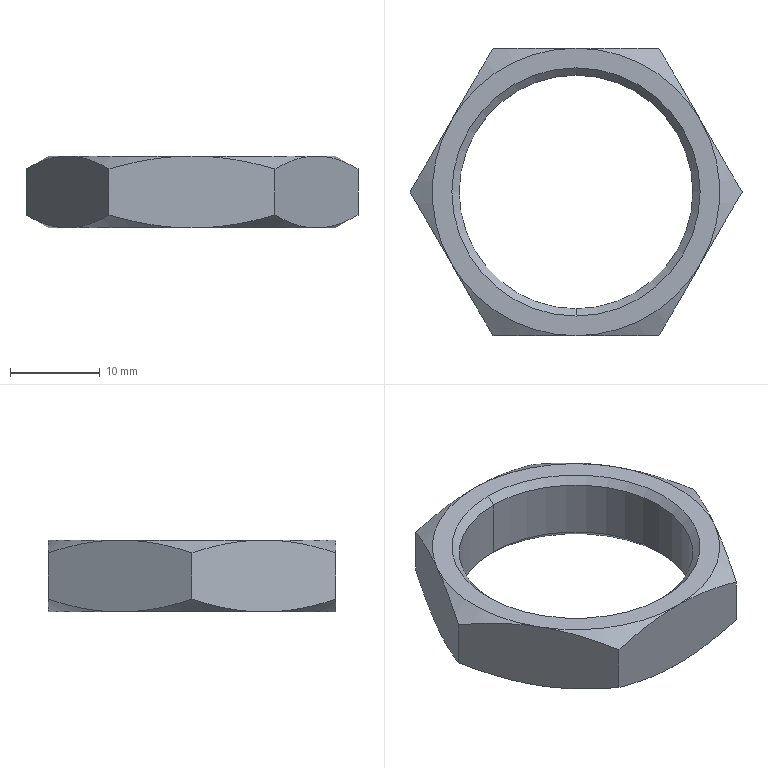Component | SolidWorks | MF_25x50_S_U_M_2_0-1_MF25_M26x1_5_Nut-1 | 1 solid | 26 faces | box 36.95 x 32 x 8 mm | volume 2721 mm3 | cone 16 | plane 8 | cylinder 2 | commonest cylinder face diameters 26 x2
build123d program:
from build123d import *

# Parameters (mm, degrees)
SKETCH2_W      = 64
SKETCH2_H      = 64
EXTRUDE1_DEPTH = 8


with BuildPart() as part:
    # Sketch1 → Revolve1 (revolve)
    with BuildSketch(Plane.XY, mode=Mode.PRIVATE) as revolve1_sk:
        Polygon((0, 0), (0, 16), (1.848, 19.2), (6.152, 19.2), (8, 16), (8, 0), align=None)
    revolve(revolve1_sk.sketch.rotate(Axis((8, 0, 0), (-1, 0, 0)), 270), axis=Axis((8, 0, 0), (-1, 0, 0)))

    # Sketch2 → Extrude1 (cut)
    with BuildSketch(Plane(origin=(0, 0, 0), x_dir=(0, 0, -1), z_dir=(1, 0, 0))):
        Rectangle(SKETCH2_W, SKETCH2_H)
        Polygon((-16, 9.238), (-16, -9.238), (0, -18.475), (16, -9.238), (16, 9.238), (0, 18.475), align=None, mode=Mode.SUBTRACT)
    extrude(amount=EXTRUDE1_DEPTH, mode=Mode.SUBTRACT)

    # Sketch3 → Cut-Revolve1 (revolve, cut)
    with BuildSketch(Plane.XY, mode=Mode.PRIVATE) as cut_revolve1_sk:
        Polygon((0, 0), (0, 13), (0.812, 12.188), (7.188, 12.188), (8, 13), (8, 0), align=None)
    revolve(cut_revolve1_sk.sketch.rotate(Axis((8, 0, 0), (-1, 0, 0)), 270), axis=Axis((8, 0, 0), (-1, 0, 0)), mode=Mode.SUBTRACT)

    # Sketch4 → Thread bore relief to major dia (revolve, cut)
    with BuildSketch(Plane.XY, mode=Mode.PRIVATE) as thread_bore_relief_to_major_dia_sk:
        Polygon((0, 0), (0, 13.812), (0.812, 13), (7.188, 13), (8, 13.812), (8, 0), align=None)
    revolve(thread_bore_relief_to_major_dia_sk.sketch.rotate(Axis((8, 0, 0), (-1, 0, 0)), 90), axis=Axis((8, 0, 0), (-1, 0, 0)), mode=Mode.SUBTRACT)


solid = part.part

# Placed as in the assembly
solid = solid.moved(Location((-102.5, -29.5, 202), (90, 0, 90)))
STEP:
#1=CARTESIAN_POINT('',(-4.035,-1.673,8.236));
#2=VERTEX_POINT('',#1);
#3=CARTESIAN_POINT('',(-4.035,-0.6496,8.236));
#4=VERTEX_POINT('',#3);
#5=CARTESIAN_POINT('',(-4.035,-1.161,8.236));
#6=DIRECTION('',(0.,0.,1.));
#7=DIRECTION('',(0.,1.,0.));
#8=AXIS2_PLACEMENT_3D('',#5,#6,#7);
#9=CIRCLE('',#8,0.5118);
#10=EDGE_CURVE('',#2,#4,#9,.T.);
#11=ORIENTED_EDGE('',*,*,#10,.F.);
#12=CARTESIAN_POINT('',(-4.035,-1.705,8.268));
#13=VERTEX_POINT('',#12);
#14=CARTESIAN_POINT('',(-4.035,-1.705,8.268));
#15=DIRECTION('',(-0.,-0.7071,0.7071));
#16=VECTOR('',#15,39.37);
#17=LINE('',#14,#16);
#18=EDGE_CURVE('',#2,#13,#17,.T.);
#19=ORIENTED_EDGE('',*,*,#18,.T.);
#20=CARTESIAN_POINT('',(-4.035,-0.6176,8.268));
#21=VERTEX_POINT('',#20);
#22=CARTESIAN_POINT('',(-4.035,-1.161,8.268));
#23=DIRECTION('',(0.,0.,1.));
#24=DIRECTION('',(0.,1.,0.));
#25=AXIS2_PLACEMENT_3D('',#22,#23,#24);
#26=CIRCLE('',#25,0.5438);
#27=EDGE_CURVE('',#13,#21,#26,.T.);
#28=ORIENTED_EDGE('',*,*,#27,.T.);
#29=CARTESIAN_POINT('',(-4.035,-0.6176,8.268));
#30=DIRECTION('',(0.,0.7071,0.7071));
#31=VECTOR('',#30,39.37);
#32=LINE('',#29,#31);
#33=EDGE_CURVE('',#4,#21,#32,.T.);
#34=ORIENTED_EDGE('',*,*,#33,.F.);
#35=EDGE_LOOP('',(#11,#19,#28,#34));
#36=FACE_OUTER_BOUND('',#35,.T.);
#37=CARTESIAN_POINT('',(-4.035,-1.161,8.268));
#38=DIRECTION('',(0.,0.,1.));
#39=DIRECTION('',(0.,1.,0.));
#40=AXIS2_PLACEMENT_3D('',#37,#38,#39);
#41=CONICAL_SURFACE('',#40,0.5438,0.7854);
#42=ADVANCED_FACE('',(#36),#41,.F.);
#43=CARTESIAN_POINT('',(-4.035,-1.673,7.985));
#44=VERTEX_POINT('',#43);
#45=CARTESIAN_POINT('',(-4.035,-0.6496,7.985));
#46=VERTEX_POINT('',#45);
#47=CARTESIAN_POINT('',(-4.035,-1.161,7.985));
#48=DIRECTION('',(0.,0.,1.));
#49=DIRECTION('',(0.,1.,0.));
#50=AXIS2_PLACEMENT_3D('',#47,#48,#49);
#51=CIRCLE('',#50,0.5118);
#52=EDGE_CURVE('',#44,#46,#51,.T.);
#53=ORIENTED_EDGE('',*,*,#52,.F.);
#54=CARTESIAN_POINT('',(-4.035,-1.673,8.268));
#55=DIRECTION('',(0.,0.,1.));
#56=VECTOR('',#55,39.37);
#57=LINE('',#54,#56);
#58=EDGE_CURVE('',#44,#2,#57,.T.);
#59=ORIENTED_EDGE('',*,*,#58,.T.);
#60=ORIENTED_EDGE('',*,*,#10,.T.);
#61=CARTESIAN_POINT('',(-4.035,-0.6496,8.268));
#62=DIRECTION('',(0.,0.,1.));
#63=VECTOR('',#62,39.37);
#64=LINE('',#61,#63);
#65=EDGE_CURVE('',#46,#4,#64,.T.);
#66=ORIENTED_EDGE('',*,*,#65,.F.);
#67=EDGE_LOOP('',(#53,#59,#60,#66));
#68=FACE_OUTER_BOUND('',#67,.T.);
#69=CARTESIAN_POINT('',(-4.035,-1.161,8.268));
#70=DIRECTION('',(0.,0.,1.));
#71=DIRECTION('',(0.,1.,0.));
#72=AXIS2_PLACEMENT_3D('',#69,#70,#71);
#73=CYLINDRICAL_SURFACE('',#72,0.5118);
#74=ADVANCED_FACE('',(#68),#73,.F.);
#75=ORIENTED_EDGE('',*,*,#52,.T.);
#76=CARTESIAN_POINT('',(-4.035,-0.6176,7.953));
#77=VERTEX_POINT('',#76);
#78=CARTESIAN_POINT('',(-4.035,-0.6496,7.985));
#79=DIRECTION('',(-0.,0.7071,-0.7071));
#80=VECTOR('',#79,39.37);
#81=LINE('',#78,#80);
#82=EDGE_CURVE('',#46,#77,#81,.T.);
#83=ORIENTED_EDGE('',*,*,#82,.T.);
#84=CARTESIAN_POINT('',(-4.035,-1.705,7.953));
#85=VERTEX_POINT('',#84);
#86=CARTESIAN_POINT('',(-4.035,-1.161,7.953));
#87=DIRECTION('',(0.,0.,1.));
#88=DIRECTION('',(0.,1.,0.));
#89=AXIS2_PLACEMENT_3D('',#86,#87,#88);
#90=CIRCLE('',#89,0.5438);
#91=EDGE_CURVE('',#85,#77,#90,.T.);
#92=ORIENTED_EDGE('',*,*,#91,.F.);
#93=CARTESIAN_POINT('',(-4.035,-1.673,7.985));
#94=DIRECTION('',(-0.,-0.7071,-0.7071));
#95=VECTOR('',#94,39.37);
#96=LINE('',#93,#95);
#97=EDGE_CURVE('',#44,#85,#96,.T.);
#98=ORIENTED_EDGE('',*,*,#97,.F.);
#99=EDGE_LOOP('',(#75,#83,#92,#98));
#100=FACE_OUTER_BOUND('',#99,.T.);
#101=CARTESIAN_POINT('',(-4.035,-1.161,7.985));
#102=DIRECTION('',(-0.,-0.,-1.));
#103=DIRECTION('',(0.,-1.,0.));
#104=AXIS2_PLACEMENT_3D('',#101,#102,#103);
#105=CONICAL_SURFACE('',#104,0.5118,0.7854);
#106=ADVANCED_FACE('',(#100),#105,.F.);
#107=ORIENTED_EDGE('',*,*,#91,.T.);
#108=CARTESIAN_POINT('',(-4.035,-1.161,7.953));
#109=DIRECTION('',(0.,0.,1.));
#110=DIRECTION('',(0.,1.,0.));
#111=AXIS2_PLACEMENT_3D('',#108,#109,#110);
#112=CIRCLE('',#111,0.5438);
#113=EDGE_CURVE('',#77,#85,#112,.T.);
#114=ORIENTED_EDGE('',*,*,#113,.T.);
#115=EDGE_LOOP('',(#107,#114));
#116=FACE_BOUND('',#115,.T.);
#117=CARTESIAN_POINT('',(-4.035,-1.791,7.953));
#118=VERTEX_POINT('',#117);
#119=CARTESIAN_POINT('',(-4.581,-1.476,7.953));
#120=VERTEX_POINT('',#119);
#121=CARTESIAN_POINT('',(-4.035,-1.161,7.953));
#122=DIRECTION('',(-0.,-0.,-1.));
#123=DIRECTION('',(0.,-1.,0.));
#124=AXIS2_PLACEMENT_3D('',#121,#122,#123);
#125=CIRCLE('',#124,0.6299);
#126=EDGE_CURVE('',#118,#120,#125,.T.);
#127=ORIENTED_EDGE('',*,*,#126,.T.);
#128=CARTESIAN_POINT('',(-4.581,-0.8465,7.953));
#129=VERTEX_POINT('',#128);
#130=CARTESIAN_POINT('',(-4.035,-1.161,7.953));
#131=DIRECTION('',(-0.,-0.,-1.));
#132=DIRECTION('',(0.,-1.,0.));
#133=AXIS2_PLACEMENT_3D('',#130,#131,#132);
#134=CIRCLE('',#133,0.6299);
#135=EDGE_CURVE('',#120,#129,#134,.T.);
#136=ORIENTED_EDGE('',*,*,#135,.T.);
#137=CARTESIAN_POINT('',(-4.035,-0.5315,7.953));
#138=VERTEX_POINT('',#137);
#139=CARTESIAN_POINT('',(-4.035,-1.161,7.953));
#140=DIRECTION('',(-0.,-0.,-1.));
#141=DIRECTION('',(0.,-1.,0.));
#142=AXIS2_PLACEMENT_3D('',#139,#140,#141);
#143=CIRCLE('',#142,0.6299);
#144=EDGE_CURVE('',#129,#138,#143,.T.);
#145=ORIENTED_EDGE('',*,*,#144,.T.);
#146=CARTESIAN_POINT('',(-3.49,-0.8465,7.953));
#147=VERTEX_POINT('',#146);
#148=CARTESIAN_POINT('',(-4.035,-1.161,7.953));
#149=DIRECTION('',(-0.,-0.,-1.));
#150=DIRECTION('',(0.,-1.,0.));
#151=AXIS2_PLACEMENT_3D('',#148,#149,#150);
#152=CIRCLE('',#151,0.6299);
#153=EDGE_CURVE('',#138,#147,#152,.T.);
#154=ORIENTED_EDGE('',*,*,#153,.T.);
#155=CARTESIAN_POINT('',(-3.49,-1.476,7.953));
#156=VERTEX_POINT('',#155);
#157=CARTESIAN_POINT('',(-4.035,-1.161,7.953));
#158=DIRECTION('',(-0.,-0.,-1.));
#159=DIRECTION('',(0.,-1.,0.));
#160=AXIS2_PLACEMENT_3D('',#157,#158,#159);
#161=CIRCLE('',#160,0.6299);
#162=EDGE_CURVE('',#147,#156,#161,.T.);
#163=ORIENTED_EDGE('',*,*,#162,.T.);
#164=CARTESIAN_POINT('',(-4.035,-1.161,7.953));
#165=DIRECTION('',(-0.,-0.,-1.));
#166=DIRECTION('',(0.,-1.,0.));
#167=AXIS2_PLACEMENT_3D('',#164,#165,#166);
#168=CIRCLE('',#167,0.6299);
#169=EDGE_CURVE('',#156,#118,#168,.T.);
#170=ORIENTED_EDGE('',*,*,#169,.T.);
#171=EDGE_LOOP('',(#127,#136,#145,#154,#163,#170));
#172=FACE_OUTER_BOUND('',#171,.T.);
#173=CARTESIAN_POINT('',(-4.035,-1.161,7.953));
#174=DIRECTION('',(0.,0.,1.));
#175=DIRECTION('',(0.,1.,-0.));
#176=AXIS2_PLACEMENT_3D('',#173,#174,#175);
#177=PLANE('',#176);
#178=ADVANCED_FACE('',(#116,#172),#177,.F.);
#179=CARTESIAN_POINT('',(-4.035,-1.161,8.268));
#180=DIRECTION('',(0.,0.,1.));
#181=DIRECTION('',(0.,1.,0.));
#182=AXIS2_PLACEMENT_3D('',#179,#180,#181);
#183=CIRCLE('',#182,0.5438);
#184=EDGE_CURVE('',#21,#13,#183,.T.);
#185=ORIENTED_EDGE('',*,*,#184,.F.);
#186=ORIENTED_EDGE('',*,*,#27,.F.);
#187=EDGE_LOOP('',(#185,#186));
#188=FACE_BOUND('',#187,.T.);
#189=CARTESIAN_POINT('',(-4.035,-1.791,8.268));
#190=VERTEX_POINT('',#189);
#191=CARTESIAN_POINT('',(-4.581,-1.476,8.268));
#192=VERTEX_POINT('',#191);
#193=CARTESIAN_POINT('',(-4.035,-1.161,8.268));
#194=DIRECTION('',(-0.,-0.,-1.));
#195=DIRECTION('',(0.,-1.,0.));
#196=AXIS2_PLACEMENT_3D('',#193,#194,#195);
#197=CIRCLE('',#196,0.6299);
#198=EDGE_CURVE('',#190,#192,#197,.T.);
#199=ORIENTED_EDGE('',*,*,#198,.F.);
#200=CARTESIAN_POINT('',(-3.49,-1.476,8.268));
#201=VERTEX_POINT('',#200);
#202=CARTESIAN_POINT('',(-4.035,-1.161,8.268));
#203=DIRECTION('',(-0.,-0.,-1.));
#204=DIRECTION('',(0.,-1.,0.));
#205=AXIS2_PLACEMENT_3D('',#202,#203,#204);
#206=CIRCLE('',#205,0.6299);
#207=EDGE_CURVE('',#201,#190,#206,.T.);
#208=ORIENTED_EDGE('',*,*,#207,.F.);
#209=CARTESIAN_POINT('',(-3.49,-0.8465,8.268));
#210=VERTEX_POINT('',#209);
#211=CARTESIAN_POINT('',(-4.035,-1.161,8.268));
#212=DIRECTION('',(-0.,-0.,-1.));
#213=DIRECTION('',(0.,-1.,0.));
#214=AXIS2_PLACEMENT_3D('',#211,#212,#213);
#215=CIRCLE('',#214,0.6299);
#216=EDGE_CURVE('',#210,#201,#215,.T.);
#217=ORIENTED_EDGE('',*,*,#216,.F.);
#218=CARTESIAN_POINT('',(-4.035,-0.5315,8.268));
#219=VERTEX_POINT('',#218);
#220=CARTESIAN_POINT('',(-4.035,-1.161,8.268));
#221=DIRECTION('',(-0.,-0.,-1.));
#222=DIRECTION('',(0.,-1.,0.));
#223=AXIS2_PLACEMENT_3D('',#220,#221,#222);
#224=CIRCLE('',#223,0.6299);
#225=EDGE_CURVE('',#219,#210,#224,.T.);
#226=ORIENTED_EDGE('',*,*,#225,.F.);
#227=CARTESIAN_POINT('',(-4.581,-0.8465,8.268));
#228=VERTEX_POINT('',#227);
#229=CARTESIAN_POINT('',(-4.035,-1.161,8.268));
#230=DIRECTION('',(-0.,-0.,-1.));
#231=DIRECTION('',(0.,-1.,0.));
#232=AXIS2_PLACEMENT_3D('',#229,#230,#231);
#233=CIRCLE('',#232,0.6299);
#234=EDGE_CURVE('',#228,#219,#233,.T.);
#235=ORIENTED_EDGE('',*,*,#234,.F.);
#236=CARTESIAN_POINT('',(-4.035,-1.161,8.268));
#237=DIRECTION('',(-0.,-0.,-1.));
#238=DIRECTION('',(0.,-1.,0.));
#239=AXIS2_PLACEMENT_3D('',#236,#237,#238);
#240=CIRCLE('',#239,0.6299);
#241=EDGE_CURVE('',#192,#228,#240,.T.);
#242=ORIENTED_EDGE('',*,*,#241,.F.);
#243=EDGE_LOOP('',(#199,#208,#217,#226,#235,#242));
#244=FACE_OUTER_BOUND('',#243,.T.);
#245=CARTESIAN_POINT('',(-4.665,-1.161,8.268));
#246=DIRECTION('',(-0.,-0.,-1.));
#247=DIRECTION('',(-0.,-1.,0.));
#248=AXIS2_PLACEMENT_3D('',#245,#246,#247);
#249=PLANE('',#248);
#250=ADVANCED_FACE('',(#188,#244),#249,.F.);
#251=CARTESIAN_POINT('',(-3.308,-1.161,8.009));
#252=VERTEX_POINT('',#251);
#253=CARTESIAN_POINT('',(-3.49,-0.8465,7.953));
#254=CARTESIAN_POINT('',(-3.474,-0.8732,7.953));
#255=CARTESIAN_POINT('',(-3.459,-0.9,7.954));
#256=CARTESIAN_POINT('',(-3.428,-0.9531,7.959));
#257=CARTESIAN_POINT('',(-3.413,-0.9795,7.963));
#258=CARTESIAN_POINT('',(-3.368,-1.058,7.978));
#259=CARTESIAN_POINT('',(-3.338,-1.11,7.992));
#260=CARTESIAN_POINT('',(-3.308,-1.161,8.009));
#261=B_SPLINE_CURVE_WITH_KNOTS('',3,(#253,#254,#255,#256,#257,#258,#259,#260),.UNSPECIFIED.,.F.,.F.,(4,2,2,4),(0.009347,0.01168,0.014,0.01866),.UNSPECIFIED.);
#262=EDGE_CURVE('',#147,#252,#261,.T.);
#263=ORIENTED_EDGE('',*,*,#262,.T.);
#264=CARTESIAN_POINT('',(-3.308,-1.161,8.009));
#265=CARTESIAN_POINT('',(-3.338,-1.213,7.992));
#266=CARTESIAN_POINT('',(-3.368,-1.265,7.978));
#267=CARTESIAN_POINT('',(-3.428,-1.37,7.958));
#268=CARTESIAN_POINT('',(-3.459,-1.423,7.953));
#269=CARTESIAN_POINT('',(-3.49,-1.476,7.953));
#270=B_SPLINE_CURVE_WITH_KNOTS('',3,(#264,#265,#266,#267,#268,#269),.UNSPECIFIED.,.F.,.F.,(4,2,4),(0.00000024,0.004674,0.009347),.UNSPECIFIED.);
#271=EDGE_CURVE('',#252,#156,#270,.T.);
#272=ORIENTED_EDGE('',*,*,#271,.T.);
#273=ORIENTED_EDGE('',*,*,#162,.F.);
#274=EDGE_LOOP('',(#263,#272,#273));
#275=FACE_OUTER_BOUND('',#274,.T.);
#276=CARTESIAN_POINT('',(-4.035,-1.161,8.025));
#277=DIRECTION('',(0.,0.,1.));
#278=DIRECTION('',(0.,1.,0.));
#279=AXIS2_PLACEMENT_3D('',#276,#277,#278);
#280=CONICAL_SURFACE('',#279,0.7559,1.047);
#281=ADVANCED_FACE('',(#275),#280,.T.);
#282=ORIENTED_EDGE('',*,*,#169,.F.);
#283=CARTESIAN_POINT('',(-3.672,-1.791,8.009));
#284=VERTEX_POINT('',#283);
#285=CARTESIAN_POINT('',(-3.49,-1.476,7.953));
#286=CARTESIAN_POINT('',(-3.505,-1.503,7.953));
#287=CARTESIAN_POINT('',(-3.521,-1.53,7.954));
#288=CARTESIAN_POINT('',(-3.552,-1.583,7.959));
#289=CARTESIAN_POINT('',(-3.567,-1.609,7.963));
#290=CARTESIAN_POINT('',(-3.612,-1.688,7.978));
#291=CARTESIAN_POINT('',(-3.642,-1.74,7.992));
#292=CARTESIAN_POINT('',(-3.672,-1.791,8.009));
#293=B_SPLINE_CURVE_WITH_KNOTS('',3,(#285,#286,#287,#288,#289,#290,#291,#292),.UNSPECIFIED.,.F.,.F.,(4,2,2,4),(0.009347,0.01168,0.014,0.01866),.UNSPECIFIED.);
#294=EDGE_CURVE('',#156,#284,#293,.T.);
#295=ORIENTED_EDGE('',*,*,#294,.T.);
#296=CARTESIAN_POINT('',(-3.672,-1.791,8.009));
#297=CARTESIAN_POINT('',(-3.701,-1.791,8.));
#298=CARTESIAN_POINT('',(-3.731,-1.791,7.993));
#299=CARTESIAN_POINT('',(-3.792,-1.791,7.979));
#300=CARTESIAN_POINT('',(-3.822,-1.791,7.973));
#301=CARTESIAN_POINT('',(-3.913,-1.791,7.958));
#302=CARTESIAN_POINT('',(-3.974,-1.791,7.953));
#303=CARTESIAN_POINT('',(-4.035,-1.791,7.953));
#304=B_SPLINE_CURVE_WITH_KNOTS('',3,(#296,#297,#298,#299,#300,#301,#302,#303),.UNSPECIFIED.,.F.,.F.,(4,2,2,4),(0.01655,0.01888,0.02122,0.02589),.UNSPECIFIED.);
#305=EDGE_CURVE('',#284,#118,#304,.T.);
#306=ORIENTED_EDGE('',*,*,#305,.T.);
#307=EDGE_LOOP('',(#282,#295,#306));
#308=FACE_OUTER_BOUND('',#307,.T.);
#309=CARTESIAN_POINT('',(-4.035,-1.161,8.025));
#310=DIRECTION('',(0.,0.,1.));
#311=DIRECTION('',(0.,1.,0.));
#312=AXIS2_PLACEMENT_3D('',#309,#310,#311);
#313=CONICAL_SURFACE('',#312,0.7559,1.047);
#314=ADVANCED_FACE('',(#308),#313,.T.);
#315=ORIENTED_EDGE('',*,*,#126,.F.);
#316=CARTESIAN_POINT('',(-4.399,-1.791,8.009));
#317=VERTEX_POINT('',#316);
#318=CARTESIAN_POINT('',(-4.035,-1.791,7.953));
#319=CARTESIAN_POINT('',(-4.066,-1.791,7.953));
#320=CARTESIAN_POINT('',(-4.097,-1.791,7.954));
#321=CARTESIAN_POINT('',(-4.159,-1.791,7.959));
#322=CARTESIAN_POINT('',(-4.19,-1.791,7.963));
#323=CARTESIAN_POINT('',(-4.281,-1.791,7.978));
#324=CARTESIAN_POINT('',(-4.34,-1.791,7.992));
#325=CARTESIAN_POINT('',(-4.399,-1.791,8.009));
#326=B_SPLINE_CURVE_WITH_KNOTS('',3,(#318,#319,#320,#321,#322,#323,#324,#325),.UNSPECIFIED.,.F.,.F.,(4,2,2,4),(0.02589,0.02823,0.03057,0.03524),.UNSPECIFIED.);
#327=EDGE_CURVE('',#118,#317,#326,.T.);
#328=ORIENTED_EDGE('',*,*,#327,.T.);
#329=CARTESIAN_POINT('',(-4.399,-1.791,8.009));
#330=CARTESIAN_POINT('',(-4.429,-1.74,7.992));
#331=CARTESIAN_POINT('',(-4.459,-1.688,7.978));
#332=CARTESIAN_POINT('',(-4.519,-1.583,7.958));
#333=CARTESIAN_POINT('',(-4.55,-1.53,7.953));
#334=CARTESIAN_POINT('',(-4.581,-1.476,7.953));
#335=B_SPLINE_CURVE_WITH_KNOTS('',3,(#329,#330,#331,#332,#333,#334),.UNSPECIFIED.,.F.,.F.,(4,2,4),(0.00000024,0.004674,0.009347),.UNSPECIFIED.);
#336=EDGE_CURVE('',#317,#120,#335,.T.);
#337=ORIENTED_EDGE('',*,*,#336,.T.);
#338=EDGE_LOOP('',(#315,#328,#337));
#339=FACE_OUTER_BOUND('',#338,.T.);
#340=CARTESIAN_POINT('',(-4.035,-1.161,8.025));
#341=DIRECTION('',(0.,0.,1.));
#342=DIRECTION('',(0.,1.,0.));
#343=AXIS2_PLACEMENT_3D('',#340,#341,#342);
#344=CONICAL_SURFACE('',#343,0.7559,1.047);
#345=ADVANCED_FACE('',(#339),#344,.T.);
#346=CARTESIAN_POINT('',(-3.672,-0.5315,8.009));
#347=VERTEX_POINT('',#346);
#348=CARTESIAN_POINT('',(-4.035,-0.5315,7.953));
#349=CARTESIAN_POINT('',(-3.974,-0.5315,7.953));
#350=CARTESIAN_POINT('',(-3.913,-0.5315,7.958));
#351=CARTESIAN_POINT('',(-3.822,-0.5315,7.973));
#352=CARTESIAN_POINT('',(-3.792,-0.5315,7.979));
#353=CARTESIAN_POINT('',(-3.731,-0.5315,7.993));
#354=CARTESIAN_POINT('',(-3.701,-0.5315,8.));
#355=CARTESIAN_POINT('',(-3.672,-0.5315,8.009));
#356=B_SPLINE_CURVE_WITH_KNOTS('',3,(#348,#349,#350,#351,#352,#353,#354,#355),.UNSPECIFIED.,.F.,.F.,(4,2,2,4),(0.04991,0.05459,0.05693,0.05927),.UNSPECIFIED.);
#357=EDGE_CURVE('',#138,#347,#356,.T.);
#358=ORIENTED_EDGE('',*,*,#357,.T.);
#359=CARTESIAN_POINT('',(-3.672,-0.5315,8.009));
#360=CARTESIAN_POINT('',(-3.642,-0.583,7.992));
#361=CARTESIAN_POINT('',(-3.612,-0.6349,7.978));
#362=CARTESIAN_POINT('',(-3.551,-0.7398,7.958));
#363=CARTESIAN_POINT('',(-3.521,-0.7928,7.953));
#364=CARTESIAN_POINT('',(-3.49,-0.8465,7.953));
#365=B_SPLINE_CURVE_WITH_KNOTS('',3,(#359,#360,#361,#362,#363,#364),.UNSPECIFIED.,.F.,.F.,(4,2,4),(0.00000024,0.004674,0.009347),.UNSPECIFIED.);
#366=EDGE_CURVE('',#347,#147,#365,.T.);
#367=ORIENTED_EDGE('',*,*,#366,.T.);
#368=ORIENTED_EDGE('',*,*,#153,.F.);
#369=EDGE_LOOP('',(#358,#367,#368));
#370=FACE_OUTER_BOUND('',#369,.T.);
#371=CARTESIAN_POINT('',(-4.035,-1.161,8.025));
#372=DIRECTION('',(0.,0.,1.));
#373=DIRECTION('',(0.,1.,0.));
#374=AXIS2_PLACEMENT_3D('',#371,#372,#373);
#375=CONICAL_SURFACE('',#374,0.7559,1.047);
#376=ADVANCED_FACE('',(#370),#375,.T.);
#377=ORIENTED_EDGE('',*,*,#135,.F.);
#378=CARTESIAN_POINT('',(-4.763,-1.161,8.009));
#379=VERTEX_POINT('',#378);
#380=CARTESIAN_POINT('',(-4.581,-1.476,7.953));
#381=CARTESIAN_POINT('',(-4.596,-1.45,7.953));
#382=CARTESIAN_POINT('',(-4.612,-1.423,7.954));
#383=CARTESIAN_POINT('',(-4.643,-1.37,7.959));
#384=CARTESIAN_POINT('',(-4.658,-1.343,7.963));
#385=CARTESIAN_POINT('',(-4.703,-1.265,7.978));
#386=CARTESIAN_POINT('',(-4.733,-1.213,7.992));
#387=CARTESIAN_POINT('',(-4.763,-1.161,8.009));
#388=B_SPLINE_CURVE_WITH_KNOTS('',3,(#380,#381,#382,#383,#384,#385,#386,#387),.UNSPECIFIED.,.F.,.F.,(4,2,2,4),(0.009347,0.01168,0.014,0.01866),.UNSPECIFIED.);
#389=EDGE_CURVE('',#120,#379,#388,.T.);
#390=ORIENTED_EDGE('',*,*,#389,.T.);
#391=CARTESIAN_POINT('',(-4.763,-1.161,8.009));
#392=CARTESIAN_POINT('',(-4.733,-1.11,7.992));
#393=CARTESIAN_POINT('',(-4.703,-1.058,7.978));
#394=CARTESIAN_POINT('',(-4.643,-0.9531,7.958));
#395=CARTESIAN_POINT('',(-4.612,-0.9001,7.953));
#396=CARTESIAN_POINT('',(-4.581,-0.8465,7.953));
#397=B_SPLINE_CURVE_WITH_KNOTS('',3,(#391,#392,#393,#394,#395,#396),.UNSPECIFIED.,.F.,.F.,(4,2,4),(0.00000024,0.004674,0.009347),.UNSPECIFIED.);
#398=EDGE_CURVE('',#379,#129,#397,.T.);
#399=ORIENTED_EDGE('',*,*,#398,.T.);
#400=EDGE_LOOP('',(#377,#390,#399));
#401=FACE_OUTER_BOUND('',#400,.T.);
#402=CARTESIAN_POINT('',(-4.035,-1.161,8.025));
#403=DIRECTION('',(0.,0.,1.));
#404=DIRECTION('',(0.,1.,0.));
#405=AXIS2_PLACEMENT_3D('',#402,#403,#404);
#406=CONICAL_SURFACE('',#405,0.7559,1.047);
#407=ADVANCED_FACE('',(#401),#406,.T.);
#408=CARTESIAN_POINT('',(-4.399,-0.5315,8.009));
#409=VERTEX_POINT('',#408);
#410=CARTESIAN_POINT('',(-4.581,-0.8465,7.953));
#411=CARTESIAN_POINT('',(-4.566,-0.8197,7.953));
#412=CARTESIAN_POINT('',(-4.55,-0.7929,7.954));
#413=CARTESIAN_POINT('',(-4.519,-0.7398,7.959));
#414=CARTESIAN_POINT('',(-4.504,-0.7134,7.963));
#415=CARTESIAN_POINT('',(-4.459,-0.6347,7.978));
#416=CARTESIAN_POINT('',(-4.429,-0.5829,7.992));
#417=CARTESIAN_POINT('',(-4.399,-0.5315,8.009));
#418=B_SPLINE_CURVE_WITH_KNOTS('',3,(#410,#411,#412,#413,#414,#415,#416,#417),.UNSPECIFIED.,.F.,.F.,(4,2,2,4),(0.009347,0.01168,0.014,0.01866),.UNSPECIFIED.);
#419=EDGE_CURVE('',#129,#409,#418,.T.);
#420=ORIENTED_EDGE('',*,*,#419,.T.);
#421=CARTESIAN_POINT('',(-4.399,-0.5315,8.009));
#422=CARTESIAN_POINT('',(-4.34,-0.5315,7.992));
#423=CARTESIAN_POINT('',(-4.281,-0.5315,7.978));
#424=CARTESIAN_POINT('',(-4.19,-0.5315,7.963));
#425=CARTESIAN_POINT('',(-4.159,-0.5315,7.959));
#426=CARTESIAN_POINT('',(-4.097,-0.5315,7.954));
#427=CARTESIAN_POINT('',(-4.066,-0.5315,7.953));
#428=CARTESIAN_POINT('',(-4.035,-0.5315,7.953));
#429=B_SPLINE_CURVE_WITH_KNOTS('',3,(#421,#422,#423,#424,#425,#426,#427,#428),.UNSPECIFIED.,.F.,.F.,(4,2,2,4),(0.04055,0.04523,0.04757,0.04991),.UNSPECIFIED.);
#430=EDGE_CURVE('',#409,#138,#429,.T.);
#431=ORIENTED_EDGE('',*,*,#430,.T.);
#432=ORIENTED_EDGE('',*,*,#144,.F.);
#433=EDGE_LOOP('',(#420,#431,#432));
#434=FACE_OUTER_BOUND('',#433,.T.);
#435=CARTESIAN_POINT('',(-4.035,-1.161,8.025));
#436=DIRECTION('',(0.,0.,1.));
#437=DIRECTION('',(0.,1.,0.));
#438=AXIS2_PLACEMENT_3D('',#435,#436,#437);
#439=CONICAL_SURFACE('',#438,0.7559,1.047);
#440=ADVANCED_FACE('',(#434),#439,.T.);
#441=CARTESIAN_POINT('',(-4.399,-1.791,8.211));
#442=VERTEX_POINT('',#441);
#443=CARTESIAN_POINT('',(-4.399,-1.791,8.268));
#444=DIRECTION('',(-0.,-0.,-1.));
#445=VECTOR('',#444,39.37);
#446=LINE('',#443,#445);
#447=EDGE_CURVE('',#442,#317,#446,.T.);
#448=ORIENTED_EDGE('',*,*,#447,.F.);
#449=CARTESIAN_POINT('',(-4.581,-1.476,8.268));
#450=CARTESIAN_POINT('',(-4.566,-1.503,8.268));
#451=CARTESIAN_POINT('',(-4.55,-1.53,8.266));
#452=CARTESIAN_POINT('',(-4.519,-1.583,8.261));
#453=CARTESIAN_POINT('',(-4.504,-1.609,8.257));
#454=CARTESIAN_POINT('',(-4.459,-1.688,8.243));
#455=CARTESIAN_POINT('',(-4.429,-1.74,8.229));
#456=CARTESIAN_POINT('',(-4.399,-1.791,8.211));
#457=B_SPLINE_CURVE_WITH_KNOTS('',3,(#449,#450,#451,#452,#453,#454,#455,#456),.UNSPECIFIED.,.F.,.F.,(4,2,2,4),(0.009347,0.01168,0.014,0.01866),.UNSPECIFIED.);
#458=EDGE_CURVE('',#192,#442,#457,.T.);
#459=ORIENTED_EDGE('',*,*,#458,.F.);
#460=CARTESIAN_POINT('',(-4.763,-1.161,8.211));
#461=VERTEX_POINT('',#460);
#462=CARTESIAN_POINT('',(-4.763,-1.161,8.211));
#463=CARTESIAN_POINT('',(-4.733,-1.213,8.229));
#464=CARTESIAN_POINT('',(-4.703,-1.265,8.243));
#465=CARTESIAN_POINT('',(-4.643,-1.37,8.262));
#466=CARTESIAN_POINT('',(-4.612,-1.423,8.268));
#467=CARTESIAN_POINT('',(-4.581,-1.476,8.268));
#468=B_SPLINE_CURVE_WITH_KNOTS('',3,(#462,#463,#464,#465,#466,#467),.UNSPECIFIED.,.F.,.F.,(4,2,4),(0.00000024,0.004674,0.009347),.UNSPECIFIED.);
#469=EDGE_CURVE('',#461,#192,#468,.T.);
#470=ORIENTED_EDGE('',*,*,#469,.F.);
#471=CARTESIAN_POINT('',(-4.763,-1.161,8.268));
#472=DIRECTION('',(-0.,-0.,-1.));
#473=VECTOR('',#472,39.37);
#474=LINE('',#471,#473);
#475=EDGE_CURVE('',#461,#379,#474,.T.);
#476=ORIENTED_EDGE('',*,*,#475,.T.);
#477=ORIENTED_EDGE('',*,*,#389,.F.);
#478=ORIENTED_EDGE('',*,*,#336,.F.);
#479=EDGE_LOOP('',(#448,#459,#470,#476,#477,#478));
#480=FACE_OUTER_BOUND('',#479,.T.);
#481=CARTESIAN_POINT('',(-4.763,-1.161,8.268));
#482=DIRECTION('',(0.866,0.5,-0.));
#483=DIRECTION('',(-0.5,0.866,-0.));
#484=AXIS2_PLACEMENT_3D('',#481,#482,#483);
#485=PLANE('',#484);
#486=ADVANCED_FACE('',(#480),#485,.F.);
#487=CARTESIAN_POINT('',(-3.672,-1.791,8.211));
#488=VERTEX_POINT('',#487);
#489=CARTESIAN_POINT('',(-3.672,-1.791,8.268));
#490=DIRECTION('',(-0.,-0.,-1.));
#491=VECTOR('',#490,39.37);
#492=LINE('',#489,#491);
#493=EDGE_CURVE('',#488,#284,#492,.T.);
#494=ORIENTED_EDGE('',*,*,#493,.F.);
#495=CARTESIAN_POINT('',(-4.035,-1.791,8.268));
#496=CARTESIAN_POINT('',(-3.974,-1.791,8.268));
#497=CARTESIAN_POINT('',(-3.913,-1.791,8.262));
#498=CARTESIAN_POINT('',(-3.822,-1.791,8.248));
#499=CARTESIAN_POINT('',(-3.792,-1.791,8.242));
#500=CARTESIAN_POINT('',(-3.731,-1.791,8.228));
#501=CARTESIAN_POINT('',(-3.701,-1.791,8.22));
#502=CARTESIAN_POINT('',(-3.672,-1.791,8.211));
#503=B_SPLINE_CURVE_WITH_KNOTS('',3,(#495,#496,#497,#498,#499,#500,#501,#502),.UNSPECIFIED.,.F.,.F.,(4,2,2,4),(0.04991,0.05459,0.05693,0.05927),.UNSPECIFIED.);
#504=EDGE_CURVE('',#190,#488,#503,.T.);
#505=ORIENTED_EDGE('',*,*,#504,.F.);
#506=CARTESIAN_POINT('',(-4.399,-1.791,8.211));
#507=CARTESIAN_POINT('',(-4.34,-1.791,8.228));
#508=CARTESIAN_POINT('',(-4.281,-1.791,8.243));
#509=CARTESIAN_POINT('',(-4.19,-1.791,8.257));
#510=CARTESIAN_POINT('',(-4.159,-1.791,8.261));
#511=CARTESIAN_POINT('',(-4.097,-1.791,8.266));
#512=CARTESIAN_POINT('',(-4.066,-1.791,8.268));
#513=CARTESIAN_POINT('',(-4.035,-1.791,8.268));
#514=B_SPLINE_CURVE_WITH_KNOTS('',3,(#506,#507,#508,#509,#510,#511,#512,#513),.UNSPECIFIED.,.F.,.F.,(4,2,2,4),(0.04055,0.04523,0.04757,0.04991),.UNSPECIFIED.);
#515=EDGE_CURVE('',#442,#190,#514,.T.);
#516=ORIENTED_EDGE('',*,*,#515,.F.);
#517=ORIENTED_EDGE('',*,*,#447,.T.);
#518=ORIENTED_EDGE('',*,*,#327,.F.);
#519=ORIENTED_EDGE('',*,*,#305,.F.);
#520=EDGE_LOOP('',(#494,#505,#516,#517,#518,#519));
#521=FACE_OUTER_BOUND('',#520,.T.);
#522=CARTESIAN_POINT('',(-4.399,-1.791,8.268));
#523=DIRECTION('',(0.,1.,-0.));
#524=DIRECTION('',(-0.,-0.,-1.));
#525=AXIS2_PLACEMENT_3D('',#522,#523,#524);
#526=PLANE('',#525);
#527=ADVANCED_FACE('',(#521),#526,.F.);
#528=CARTESIAN_POINT('',(-3.308,-1.161,8.211));
#529=VERTEX_POINT('',#528);
#530=CARTESIAN_POINT('',(-3.308,-1.161,8.268));
#531=DIRECTION('',(-0.,-0.,-1.));
#532=VECTOR('',#531,39.37);
#533=LINE('',#530,#532);
#534=EDGE_CURVE('',#529,#252,#533,.T.);
#535=ORIENTED_EDGE('',*,*,#534,.F.);
#536=CARTESIAN_POINT('',(-3.49,-1.476,8.268));
#537=CARTESIAN_POINT('',(-3.474,-1.45,8.268));
#538=CARTESIAN_POINT('',(-3.459,-1.423,8.266));
#539=CARTESIAN_POINT('',(-3.428,-1.37,8.261));
#540=CARTESIAN_POINT('',(-3.413,-1.343,8.257));
#541=CARTESIAN_POINT('',(-3.368,-1.265,8.243));
#542=CARTESIAN_POINT('',(-3.338,-1.213,8.229));
#543=CARTESIAN_POINT('',(-3.308,-1.161,8.211));
#544=B_SPLINE_CURVE_WITH_KNOTS('',3,(#536,#537,#538,#539,#540,#541,#542,#543),.UNSPECIFIED.,.F.,.F.,(4,2,2,4),(0.009347,0.01168,0.014,0.01866),.UNSPECIFIED.);
#545=EDGE_CURVE('',#201,#529,#544,.T.);
#546=ORIENTED_EDGE('',*,*,#545,.F.);
#547=CARTESIAN_POINT('',(-3.672,-1.791,8.211));
#548=CARTESIAN_POINT('',(-3.642,-1.74,8.229));
#549=CARTESIAN_POINT('',(-3.612,-1.688,8.243));
#550=CARTESIAN_POINT('',(-3.551,-1.583,8.262));
#551=CARTESIAN_POINT('',(-3.521,-1.53,8.268));
#552=CARTESIAN_POINT('',(-3.49,-1.476,8.268));
#553=B_SPLINE_CURVE_WITH_KNOTS('',3,(#547,#548,#549,#550,#551,#552),.UNSPECIFIED.,.F.,.F.,(4,2,4),(0.00000024,0.004674,0.009347),.UNSPECIFIED.);
#554=EDGE_CURVE('',#488,#201,#553,.T.);
#555=ORIENTED_EDGE('',*,*,#554,.F.);
#556=ORIENTED_EDGE('',*,*,#493,.T.);
#557=ORIENTED_EDGE('',*,*,#294,.F.);
#558=ORIENTED_EDGE('',*,*,#271,.F.);
#559=EDGE_LOOP('',(#535,#546,#555,#556,#557,#558));
#560=FACE_OUTER_BOUND('',#559,.T.);
#561=CARTESIAN_POINT('',(-3.672,-1.791,8.268));
#562=DIRECTION('',(-0.866,0.5,0.));
#563=DIRECTION('',(-0.5,-0.866,0.));
#564=AXIS2_PLACEMENT_3D('',#561,#562,#563);
#565=PLANE('',#564);
#566=ADVANCED_FACE('',(#560),#565,.F.);
#567=CARTESIAN_POINT('',(-3.672,-0.5315,8.211));
#568=VERTEX_POINT('',#567);
#569=CARTESIAN_POINT('',(-3.672,-0.5315,8.268));
#570=DIRECTION('',(-0.,-0.,-1.));
#571=VECTOR('',#570,39.37);
#572=LINE('',#569,#571);
#573=EDGE_CURVE('',#568,#347,#572,.T.);
#574=ORIENTED_EDGE('',*,*,#573,.F.);
#575=CARTESIAN_POINT('',(-3.49,-0.8465,8.268));
#576=CARTESIAN_POINT('',(-3.505,-0.8197,8.268));
#577=CARTESIAN_POINT('',(-3.521,-0.7929,8.266));
#578=CARTESIAN_POINT('',(-3.552,-0.7398,8.261));
#579=CARTESIAN_POINT('',(-3.567,-0.7134,8.257));
#580=CARTESIAN_POINT('',(-3.612,-0.6347,8.243));
#581=CARTESIAN_POINT('',(-3.642,-0.5829,8.229));
#582=CARTESIAN_POINT('',(-3.672,-0.5315,8.211));
#583=B_SPLINE_CURVE_WITH_KNOTS('',3,(#575,#576,#577,#578,#579,#580,#581,#582),.UNSPECIFIED.,.F.,.F.,(4,2,2,4),(0.009347,0.01168,0.014,0.01866),.UNSPECIFIED.);
#584=EDGE_CURVE('',#210,#568,#583,.T.);
#585=ORIENTED_EDGE('',*,*,#584,.F.);
#586=CARTESIAN_POINT('',(-3.308,-1.161,8.211));
#587=CARTESIAN_POINT('',(-3.338,-1.11,8.229));
#588=CARTESIAN_POINT('',(-3.368,-1.058,8.243));
#589=CARTESIAN_POINT('',(-3.428,-0.9531,8.262));
#590=CARTESIAN_POINT('',(-3.459,-0.9001,8.268));
#591=CARTESIAN_POINT('',(-3.49,-0.8465,8.268));
#592=B_SPLINE_CURVE_WITH_KNOTS('',3,(#586,#587,#588,#589,#590,#591),.UNSPECIFIED.,.F.,.F.,(4,2,4),(0.00000024,0.004674,0.009347),.UNSPECIFIED.);
#593=EDGE_CURVE('',#529,#210,#592,.T.);
#594=ORIENTED_EDGE('',*,*,#593,.F.);
#595=ORIENTED_EDGE('',*,*,#534,.T.);
#596=ORIENTED_EDGE('',*,*,#262,.F.);
#597=ORIENTED_EDGE('',*,*,#366,.F.);
#598=EDGE_LOOP('',(#574,#585,#594,#595,#596,#597));
#599=FACE_OUTER_BOUND('',#598,.T.);
#600=CARTESIAN_POINT('',(-3.308,-1.161,8.268));
#601=DIRECTION('',(-0.866,-0.5,0.));
#602=DIRECTION('',(0.5,-0.866,0.));
#603=AXIS2_PLACEMENT_3D('',#600,#601,#602);
#604=PLANE('',#603);
#605=ADVANCED_FACE('',(#599),#604,.F.);
#606=CARTESIAN_POINT('',(-4.399,-0.5315,8.211));
#607=VERTEX_POINT('',#606);
#608=CARTESIAN_POINT('',(-4.399,-0.5315,8.268));
#609=DIRECTION('',(-0.,-0.,-1.));
#610=VECTOR('',#609,39.37);
#611=LINE('',#608,#610);
#612=EDGE_CURVE('',#607,#409,#611,.T.);
#613=ORIENTED_EDGE('',*,*,#612,.F.);
#614=CARTESIAN_POINT('',(-4.035,-0.5315,8.268));
#615=CARTESIAN_POINT('',(-4.066,-0.5315,8.268));
#616=CARTESIAN_POINT('',(-4.097,-0.5315,8.266));
#617=CARTESIAN_POINT('',(-4.159,-0.5315,8.261));
#618=CARTESIAN_POINT('',(-4.19,-0.5315,8.257));
#619=CARTESIAN_POINT('',(-4.281,-0.5315,8.243));
#620=CARTESIAN_POINT('',(-4.34,-0.5315,8.228));
#621=CARTESIAN_POINT('',(-4.399,-0.5315,8.211));
#622=B_SPLINE_CURVE_WITH_KNOTS('',3,(#614,#615,#616,#617,#618,#619,#620,#621),.UNSPECIFIED.,.F.,.F.,(4,2,2,4),(0.02589,0.02823,0.03057,0.03524),.UNSPECIFIED.);
#623=EDGE_CURVE('',#219,#607,#622,.T.);
#624=ORIENTED_EDGE('',*,*,#623,.F.);
#625=CARTESIAN_POINT('',(-3.672,-0.5315,8.211));
#626=CARTESIAN_POINT('',(-3.701,-0.5315,8.22));
#627=CARTESIAN_POINT('',(-3.731,-0.5315,8.228));
#628=CARTESIAN_POINT('',(-3.792,-0.5315,8.242));
#629=CARTESIAN_POINT('',(-3.822,-0.5315,8.248));
#630=CARTESIAN_POINT('',(-3.913,-0.5315,8.262));
#631=CARTESIAN_POINT('',(-3.974,-0.5315,8.268));
#632=CARTESIAN_POINT('',(-4.035,-0.5315,8.268));
#633=B_SPLINE_CURVE_WITH_KNOTS('',3,(#625,#626,#627,#628,#629,#630,#631,#632),.UNSPECIFIED.,.F.,.F.,(4,2,2,4),(0.01655,0.01888,0.02122,0.02589),.UNSPECIFIED.);
#634=EDGE_CURVE('',#568,#219,#633,.T.);
#635=ORIENTED_EDGE('',*,*,#634,.F.);
#636=ORIENTED_EDGE('',*,*,#573,.T.);
#637=ORIENTED_EDGE('',*,*,#357,.F.);
#638=ORIENTED_EDGE('',*,*,#430,.F.);
#639=EDGE_LOOP('',(#613,#624,#635,#636,#637,#638));
#640=FACE_OUTER_BOUND('',#639,.T.);
#641=CARTESIAN_POINT('',(-3.672,-0.5315,8.268));
#642=DIRECTION('',(-0.,-1.,0.));
#643=DIRECTION('',(0.,0.,1.));
#644=AXIS2_PLACEMENT_3D('',#641,#642,#643);
#645=PLANE('',#644);
#646=ADVANCED_FACE('',(#640),#645,.F.);
#647=ORIENTED_EDGE('',*,*,#475,.F.);
#648=CARTESIAN_POINT('',(-4.581,-0.8465,8.268));
#649=CARTESIAN_POINT('',(-4.596,-0.8732,8.268));
#650=CARTESIAN_POINT('',(-4.612,-0.9,8.266));
#651=CARTESIAN_POINT('',(-4.643,-0.9531,8.261));
#652=CARTESIAN_POINT('',(-4.658,-0.9795,8.257));
#653=CARTESIAN_POINT('',(-4.703,-1.058,8.243));
#654=CARTESIAN_POINT('',(-4.733,-1.11,8.229));
#655=CARTESIAN_POINT('',(-4.763,-1.161,8.211));
#656=B_SPLINE_CURVE_WITH_KNOTS('',3,(#648,#649,#650,#651,#652,#653,#654,#655),.UNSPECIFIED.,.F.,.F.,(4,2,2,4),(0.009347,0.01168,0.014,0.01866),.UNSPECIFIED.);
#657=EDGE_CURVE('',#228,#461,#656,.T.);
#658=ORIENTED_EDGE('',*,*,#657,.F.);
#659=CARTESIAN_POINT('',(-4.399,-0.5315,8.211));
#660=CARTESIAN_POINT('',(-4.429,-0.583,8.229));
#661=CARTESIAN_POINT('',(-4.459,-0.6349,8.243));
#662=CARTESIAN_POINT('',(-4.519,-0.7398,8.262));
#663=CARTESIAN_POINT('',(-4.55,-0.7928,8.268));
#664=CARTESIAN_POINT('',(-4.581,-0.8465,8.268));
#665=B_SPLINE_CURVE_WITH_KNOTS('',3,(#659,#660,#661,#662,#663,#664),.UNSPECIFIED.,.F.,.F.,(4,2,4),(0.00000024,0.004674,0.009347),.UNSPECIFIED.);
#666=EDGE_CURVE('',#607,#228,#665,.T.);
#667=ORIENTED_EDGE('',*,*,#666,.F.);
#668=ORIENTED_EDGE('',*,*,#612,.T.);
#669=ORIENTED_EDGE('',*,*,#419,.F.);
#670=ORIENTED_EDGE('',*,*,#398,.F.);
#671=EDGE_LOOP('',(#647,#658,#667,#668,#669,#670));
#672=FACE_OUTER_BOUND('',#671,.T.);
#673=CARTESIAN_POINT('',(-4.399,-0.5315,8.268));
#674=DIRECTION('',(0.866,-0.5,-0.));
#675=DIRECTION('',(0.5,0.866,-0.));
#676=AXIS2_PLACEMENT_3D('',#673,#674,#675);
#677=PLANE('',#676);
#678=ADVANCED_FACE('',(#672),#677,.F.);
#679=ORIENTED_EDGE('',*,*,#234,.T.);
#680=ORIENTED_EDGE('',*,*,#623,.T.);
#681=ORIENTED_EDGE('',*,*,#666,.T.);
#682=EDGE_LOOP('',(#679,#680,#681));
#683=FACE_OUTER_BOUND('',#682,.T.);
#684=CARTESIAN_POINT('',(-4.035,-1.161,8.268));
#685=DIRECTION('',(-0.,-0.,-1.));
#686=DIRECTION('',(0.,-1.,0.));
#687=AXIS2_PLACEMENT_3D('',#684,#685,#686);
#688=CONICAL_SURFACE('',#687,0.6299,1.047);
#689=ADVANCED_FACE('',(#683),#688,.T.);
#690=ORIENTED_EDGE('',*,*,#225,.T.);
#691=ORIENTED_EDGE('',*,*,#584,.T.);
#692=ORIENTED_EDGE('',*,*,#634,.T.);
#693=EDGE_LOOP('',(#690,#691,#692));
#694=FACE_OUTER_BOUND('',#693,.T.);
#695=CARTESIAN_POINT('',(-4.035,-1.161,8.268));
#696=DIRECTION('',(-0.,-0.,-1.));
#697=DIRECTION('',(0.,-1.,0.));
#698=AXIS2_PLACEMENT_3D('',#695,#696,#697);
#699=CONICAL_SURFACE('',#698,0.6299,1.047);
#700=ADVANCED_FACE('',(#694),#699,.T.);
#701=ORIENTED_EDGE('',*,*,#216,.T.);
#702=ORIENTED_EDGE('',*,*,#545,.T.);
#703=ORIENTED_EDGE('',*,*,#593,.T.);
#704=EDGE_LOOP('',(#701,#702,#703));
#705=FACE_OUTER_BOUND('',#704,.T.);
#706=CARTESIAN_POINT('',(-4.035,-1.161,8.268));
#707=DIRECTION('',(-0.,-0.,-1.));
#708=DIRECTION('',(0.,-1.,0.));
#709=AXIS2_PLACEMENT_3D('',#706,#707,#708);
#710=CONICAL_SURFACE('',#709,0.6299,1.047);
#711=ADVANCED_FACE('',(#705),#710,.T.);
#712=ORIENTED_EDGE('',*,*,#207,.T.);
#713=ORIENTED_EDGE('',*,*,#504,.T.);
#714=ORIENTED_EDGE('',*,*,#554,.T.);
#715=EDGE_LOOP('',(#712,#713,#714));
#716=FACE_OUTER_BOUND('',#715,.T.);
#717=CARTESIAN_POINT('',(-4.035,-1.161,8.268));
#718=DIRECTION('',(-0.,-0.,-1.));
#719=DIRECTION('',(0.,-1.,0.));
#720=AXIS2_PLACEMENT_3D('',#717,#718,#719);
#721=CONICAL_SURFACE('',#720,0.6299,1.047);
#722=ADVANCED_FACE('',(#716),#721,.T.);
#723=ORIENTED_EDGE('',*,*,#198,.T.);
#724=ORIENTED_EDGE('',*,*,#458,.T.);
#725=ORIENTED_EDGE('',*,*,#515,.T.);
#726=EDGE_LOOP('',(#723,#724,#725));
#727=FACE_OUTER_BOUND('',#726,.T.);
#728=CARTESIAN_POINT('',(-4.035,-1.161,8.268));
#729=DIRECTION('',(-0.,-0.,-1.));
#730=DIRECTION('',(0.,-1.,0.));
#731=AXIS2_PLACEMENT_3D('',#728,#729,#730);
#732=CONICAL_SURFACE('',#731,0.6299,1.047);
#733=ADVANCED_FACE('',(#727),#732,.T.);
#734=ORIENTED_EDGE('',*,*,#657,.T.);
#735=ORIENTED_EDGE('',*,*,#469,.T.);
#736=ORIENTED_EDGE('',*,*,#241,.T.);
#737=EDGE_LOOP('',(#734,#735,#736));
#738=FACE_OUTER_BOUND('',#737,.T.);
#739=CARTESIAN_POINT('',(-4.035,-1.161,8.268));
#740=DIRECTION('',(-0.,-0.,-1.));
#741=DIRECTION('',(0.,-1.,0.));
#742=AXIS2_PLACEMENT_3D('',#739,#740,#741);
#743=CONICAL_SURFACE('',#742,0.6299,1.047);
#744=ADVANCED_FACE('',(#738),#743,.T.);
#745=ORIENTED_EDGE('',*,*,#82,.F.);
#746=CARTESIAN_POINT('',(-4.035,-1.161,7.985));
#747=DIRECTION('',(0.,0.,1.));
#748=DIRECTION('',(0.,1.,0.));
#749=AXIS2_PLACEMENT_3D('',#746,#747,#748);
#750=CIRCLE('',#749,0.5118);
#751=EDGE_CURVE('',#46,#44,#750,.T.);
#752=ORIENTED_EDGE('',*,*,#751,.T.);
#753=ORIENTED_EDGE('',*,*,#97,.T.);
#754=ORIENTED_EDGE('',*,*,#113,.F.);
#755=EDGE_LOOP('',(#745,#752,#753,#754));
#756=FACE_OUTER_BOUND('',#755,.T.);
#757=CARTESIAN_POINT('',(-4.035,-1.161,7.985));
#758=DIRECTION('',(-0.,-0.,-1.));
#759=DIRECTION('',(0.,-1.,0.));
#760=AXIS2_PLACEMENT_3D('',#757,#758,#759);
#761=CONICAL_SURFACE('',#760,0.5118,0.7854);
#762=ADVANCED_FACE('',(#756),#761,.F.);
#763=ORIENTED_EDGE('',*,*,#58,.F.);
#764=ORIENTED_EDGE('',*,*,#751,.F.);
#765=ORIENTED_EDGE('',*,*,#65,.T.);
#766=CARTESIAN_POINT('',(-4.035,-1.161,8.236));
#767=DIRECTION('',(0.,0.,1.));
#768=DIRECTION('',(0.,1.,0.));
#769=AXIS2_PLACEMENT_3D('',#766,#767,#768);
#770=CIRCLE('',#769,0.5118);
#771=EDGE_CURVE('',#4,#2,#770,.T.);
#772=ORIENTED_EDGE('',*,*,#771,.T.);
#773=EDGE_LOOP('',(#763,#764,#765,#772));
#774=FACE_OUTER_BOUND('',#773,.T.);
#775=CARTESIAN_POINT('',(-4.035,-1.161,8.268));
#776=DIRECTION('',(0.,0.,1.));
#777=DIRECTION('',(0.,1.,0.));
#778=AXIS2_PLACEMENT_3D('',#775,#776,#777);
#779=CYLINDRICAL_SURFACE('',#778,0.5118);
#780=ADVANCED_FACE('',(#774),#779,.F.);
#781=ORIENTED_EDGE('',*,*,#18,.F.);
#782=ORIENTED_EDGE('',*,*,#771,.F.);
#783=ORIENTED_EDGE('',*,*,#33,.T.);
#784=ORIENTED_EDGE('',*,*,#184,.T.);
#785=EDGE_LOOP('',(#781,#782,#783,#784));
#786=FACE_OUTER_BOUND('',#785,.T.);
#787=CARTESIAN_POINT('',(-4.035,-1.161,8.268));
#788=DIRECTION('',(0.,0.,1.));
#789=DIRECTION('',(0.,1.,0.));
#790=AXIS2_PLACEMENT_3D('',#787,#788,#789);
#791=CONICAL_SURFACE('',#790,0.5438,0.7854);
#792=ADVANCED_FACE('',(#786),#791,.F.);
#793=CLOSED_SHELL('',(#42,#74,#106,#178,#250,#281,#314,#345,#376,#407,#440,#486,#527,#566,#605,#646,#678,#689,#700,#711,#722,#733,#744,#762,#780,#792));
#794=MANIFOLD_SOLID_BREP('',#793);
#795=CARTESIAN_POINT('',(0.,0.,0.));
#796=DIRECTION('',(0.,0.,1.));
#797=DIRECTION('',(1.,0.,0.));
#798=AXIS2_PLACEMENT_3D('',#795,#796,#797);
#799=(LENGTH_UNIT()NAMED_UNIT(*)SI_UNIT($,.METRE.));
#800=LENGTH_MEASURE_WITH_UNIT(LENGTH_MEASURE(0.0254),#799);
#801=DIMENSIONAL_EXPONENTS(1.,0.,0.,0.,0.,0.,0.);
#802=(CONVERSION_BASED_UNIT('',#800)LENGTH_UNIT()NAMED_UNIT(#801));
#803=UNCERTAINTY_MEASURE_WITH_UNIT(LENGTH_MEASURE(0.00001),#802,'','');
#804=(NAMED_UNIT(*)PLANE_ANGLE_UNIT()SI_UNIT($,.RADIAN.));
#805=(NAMED_UNIT(*)SI_UNIT($,.STERADIAN.)SOLID_ANGLE_UNIT());
#806=(GEOMETRIC_REPRESENTATION_CONTEXT(3)GLOBAL_UNCERTAINTY_ASSIGNED_CONTEXT((#803))GLOBAL_UNIT_ASSIGNED_CONTEXT((#802,#804,#805))REPRESENTATION_CONTEXT('',''));
#807=ADVANCED_BREP_SHAPE_REPRESENTATION('',(#794,#798),#806);
#808=COLOUR_RGB('',0.7922,0.8196,0.9333);
#809=FILL_AREA_STYLE_COLOUR('',#808);
#810=FILL_AREA_STYLE('',(#809));
#811=SURFACE_STYLE_FILL_AREA(#810);
#812=SURFACE_SIDE_STYLE('',(#811));
#813=SURFACE_STYLE_USAGE(.BOTH.,#812);
#814=PRESENTATION_STYLE_ASSIGNMENT((#813));
#815=STYLED_ITEM('',(#814),#794);
#816=(LENGTH_UNIT()NAMED_UNIT(*)SI_UNIT($,.METRE.));
#817=LENGTH_MEASURE_WITH_UNIT(LENGTH_MEASURE(0.0254),#816);
#818=DIMENSIONAL_EXPONENTS(1.,0.,0.,0.,0.,0.,0.);
#819=(CONVERSION_BASED_UNIT('',#817)LENGTH_UNIT()NAMED_UNIT(#818));
#820=UNCERTAINTY_MEASURE_WITH_UNIT(LENGTH_MEASURE(0.00001),#819,'','');
#821=(NAMED_UNIT(*)PLANE_ANGLE_UNIT()SI_UNIT($,.RADIAN.));
#822=(NAMED_UNIT(*)SI_UNIT($,.STERADIAN.)SOLID_ANGLE_UNIT());
#823=(GEOMETRIC_REPRESENTATION_CONTEXT(3)GLOBAL_UNCERTAINTY_ASSIGNED_CONTEXT((#820))GLOBAL_UNIT_ASSIGNED_CONTEXT((#819,#821,#822))REPRESENTATION_CONTEXT('',''));
#824=MECHANICAL_DESIGN_GEOMETRIC_PRESENTATION_REPRESENTATION('',(#815),#823);
#825=PRESENTATION_LAYER_ASSIGNMENT('','',(#815));